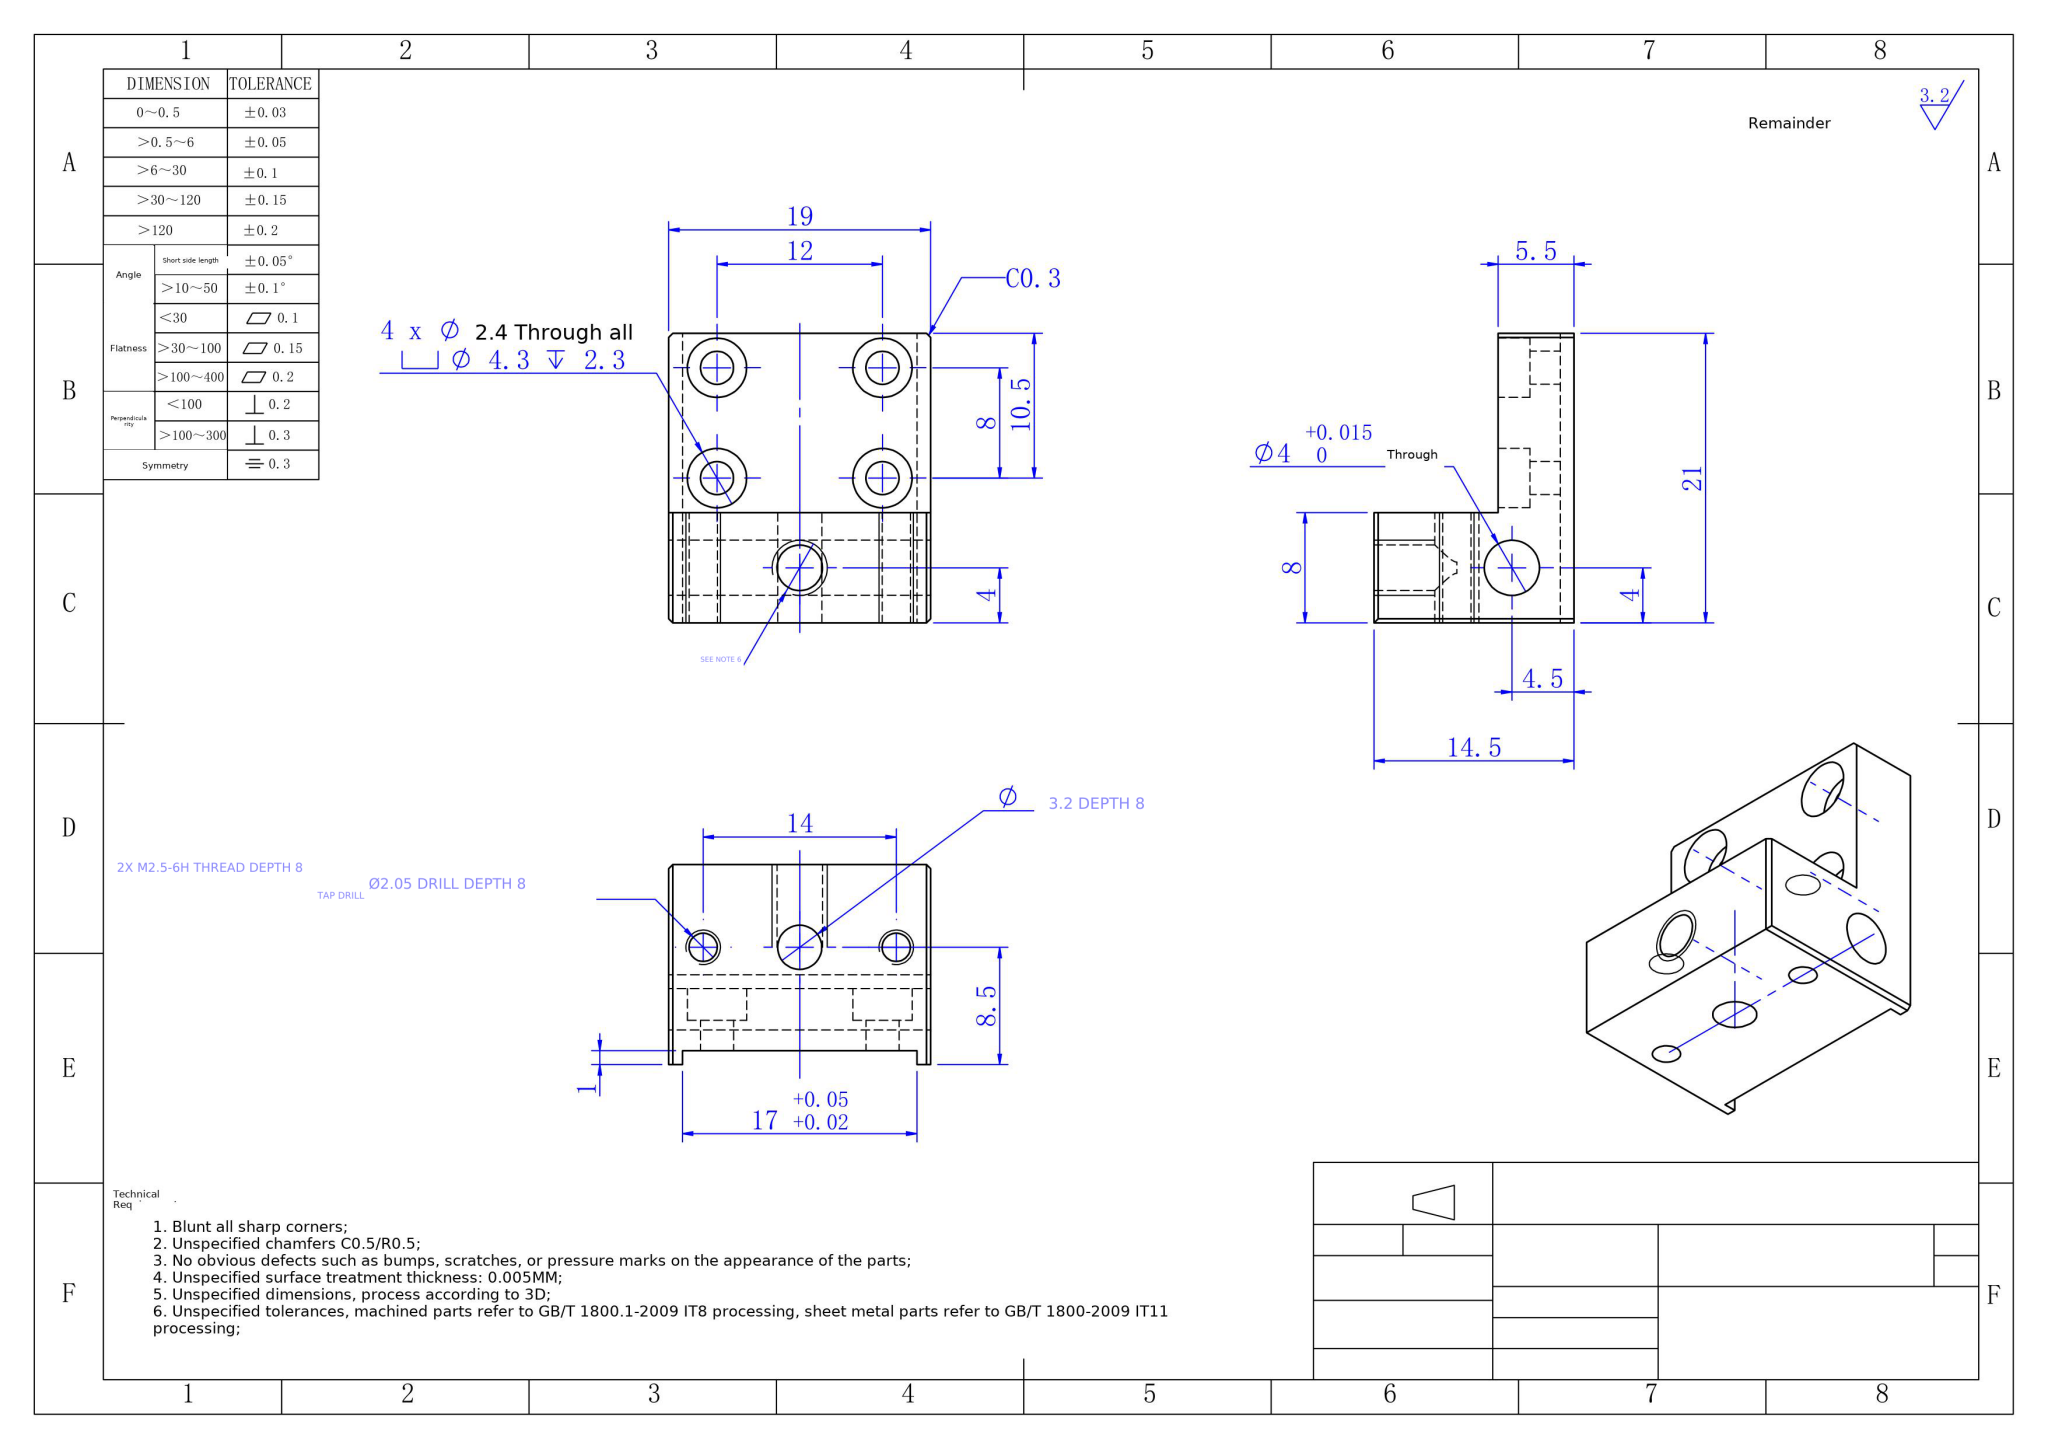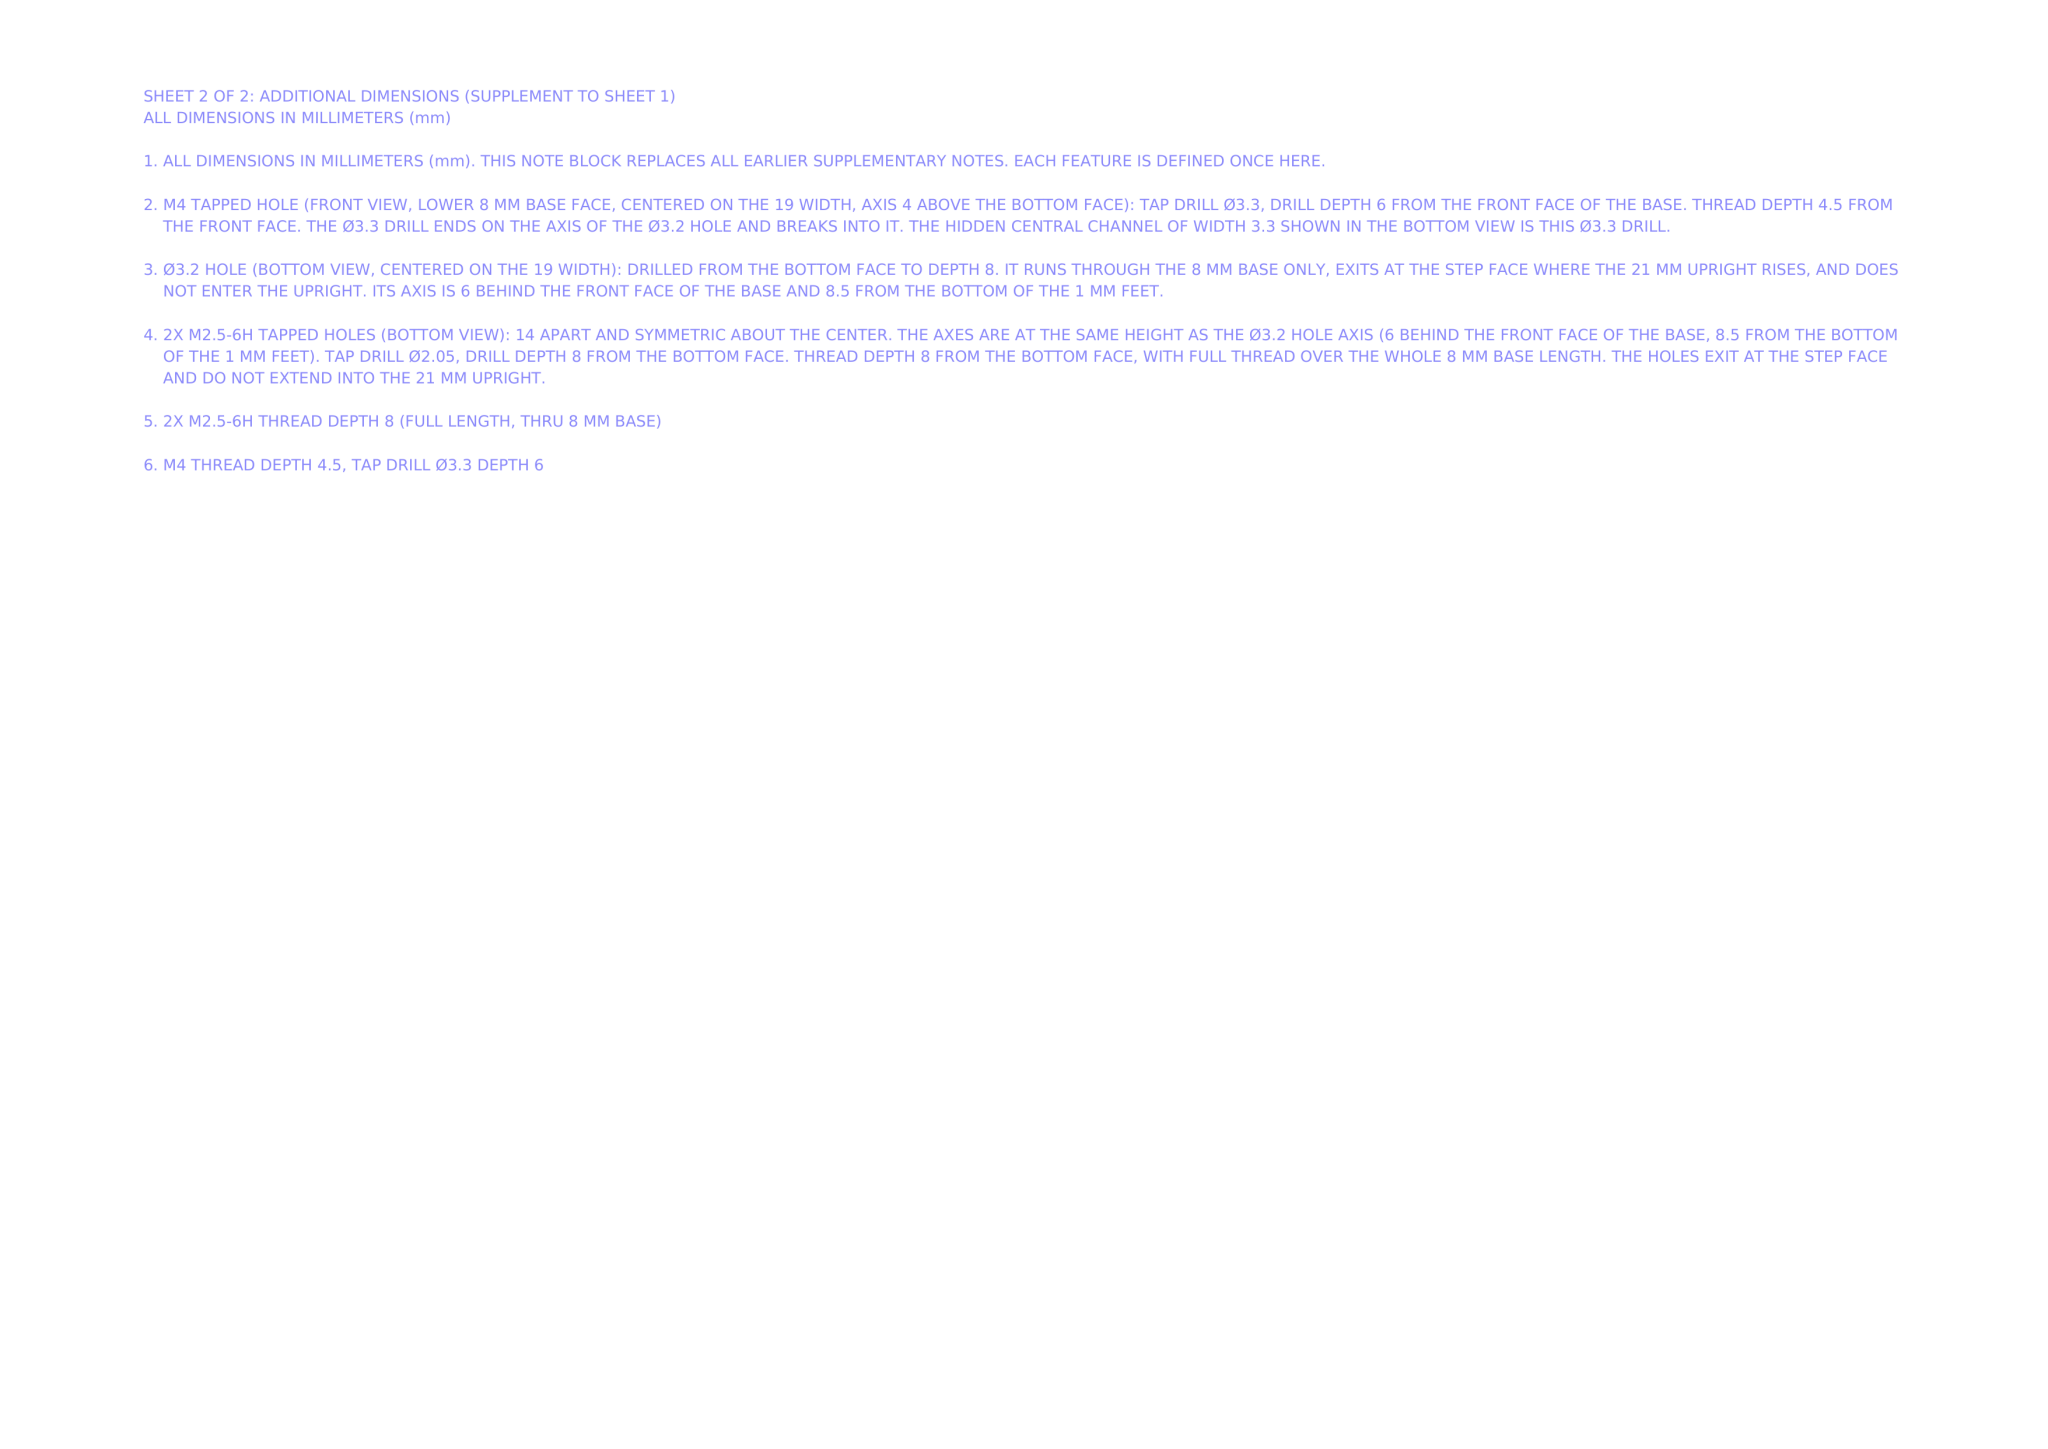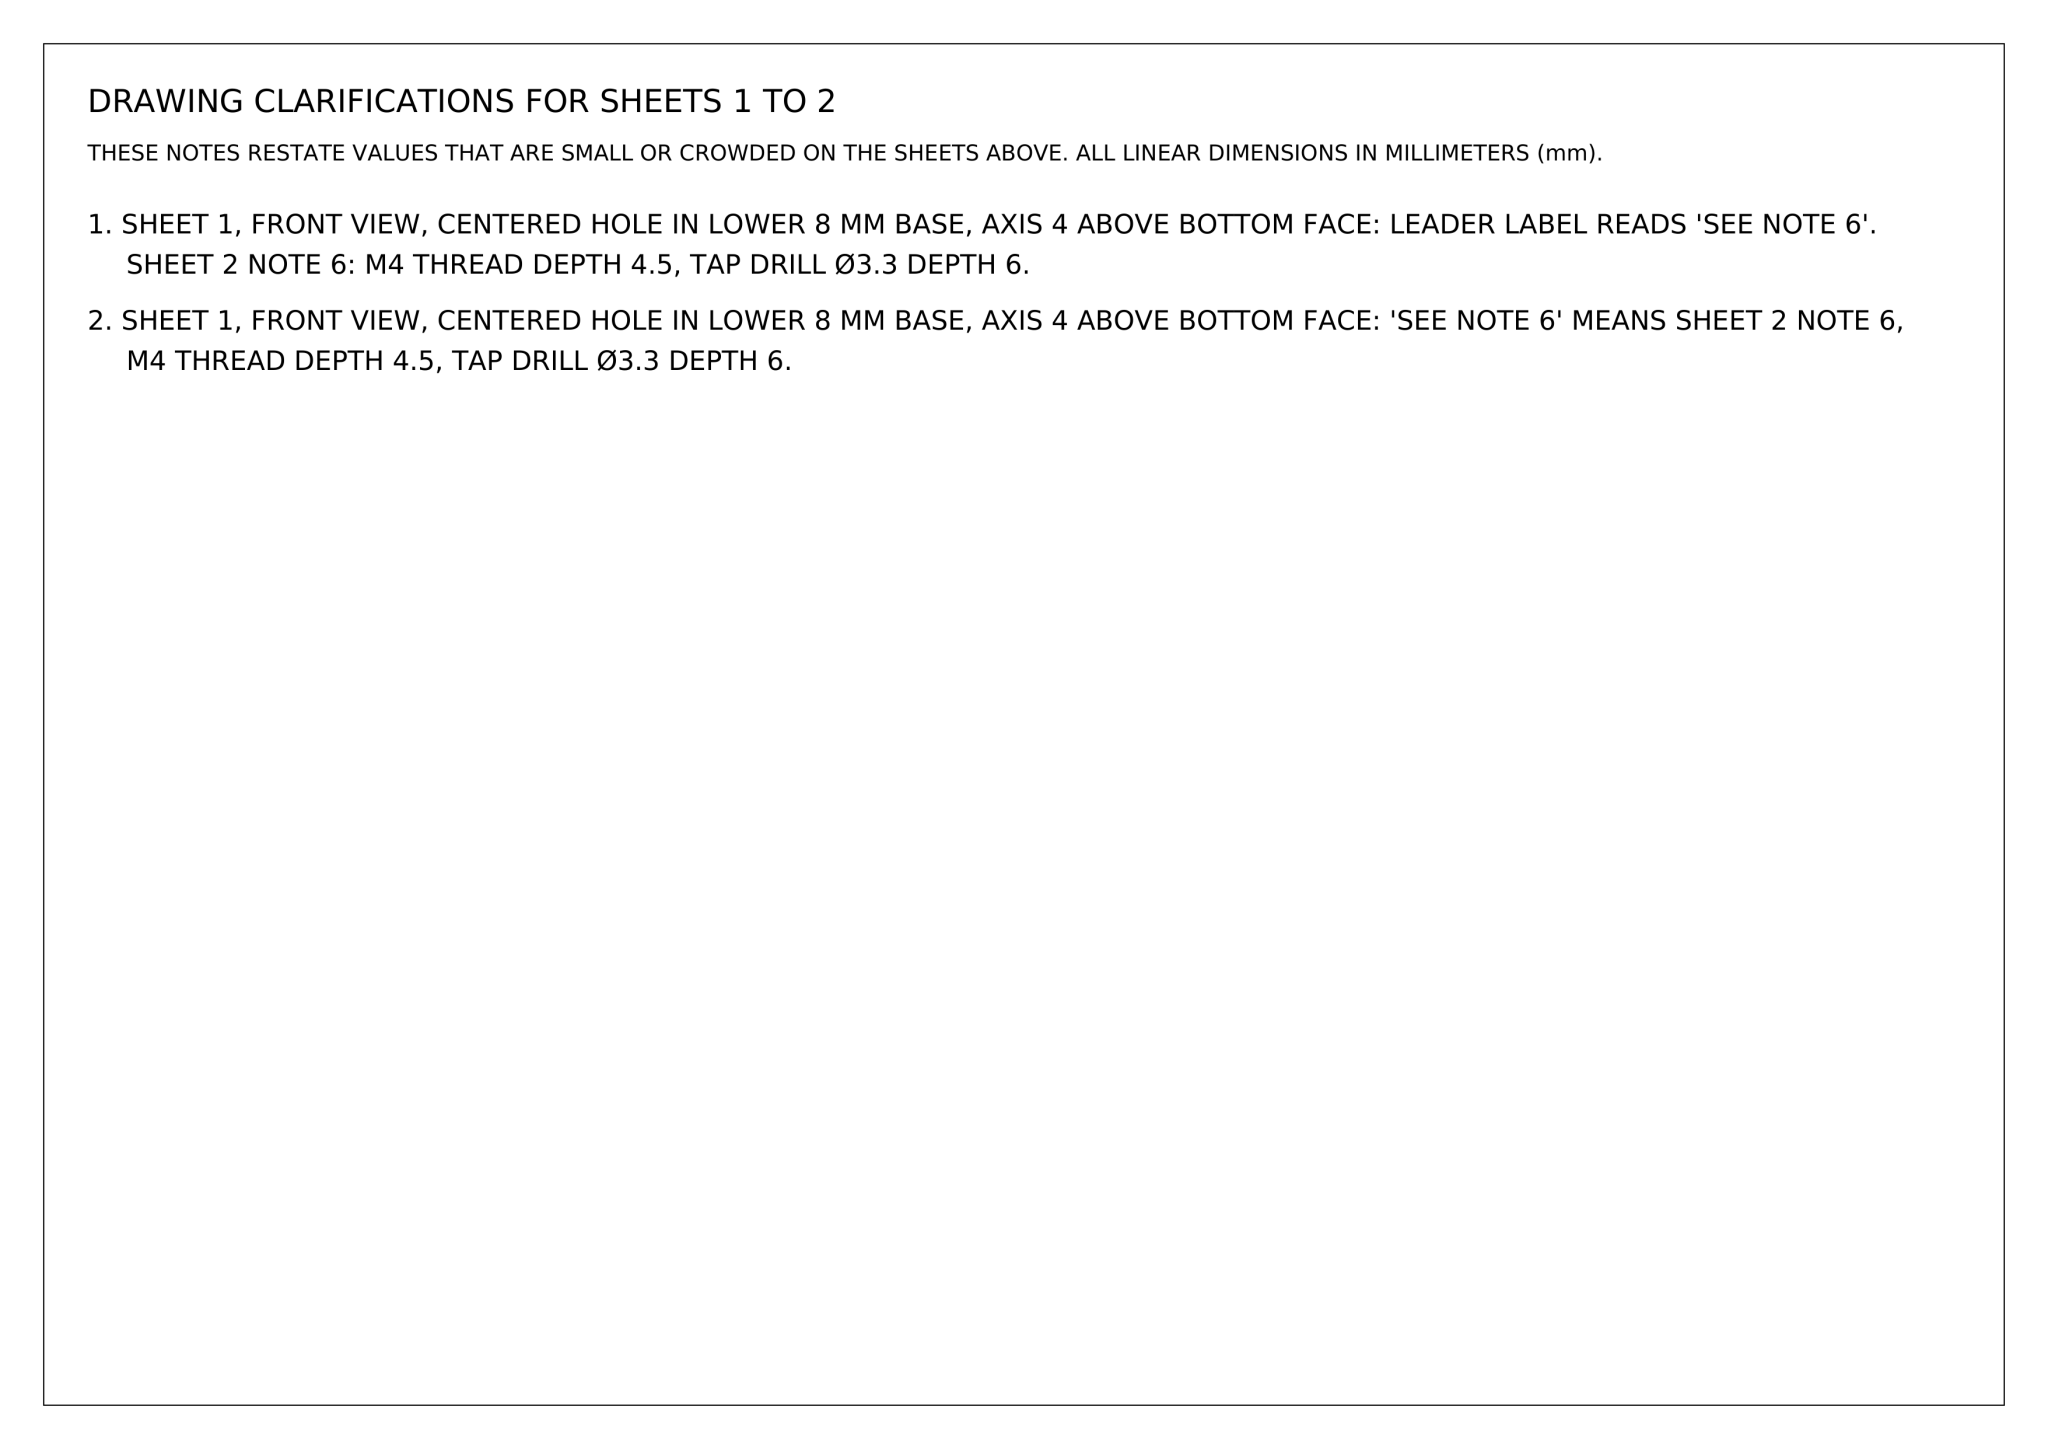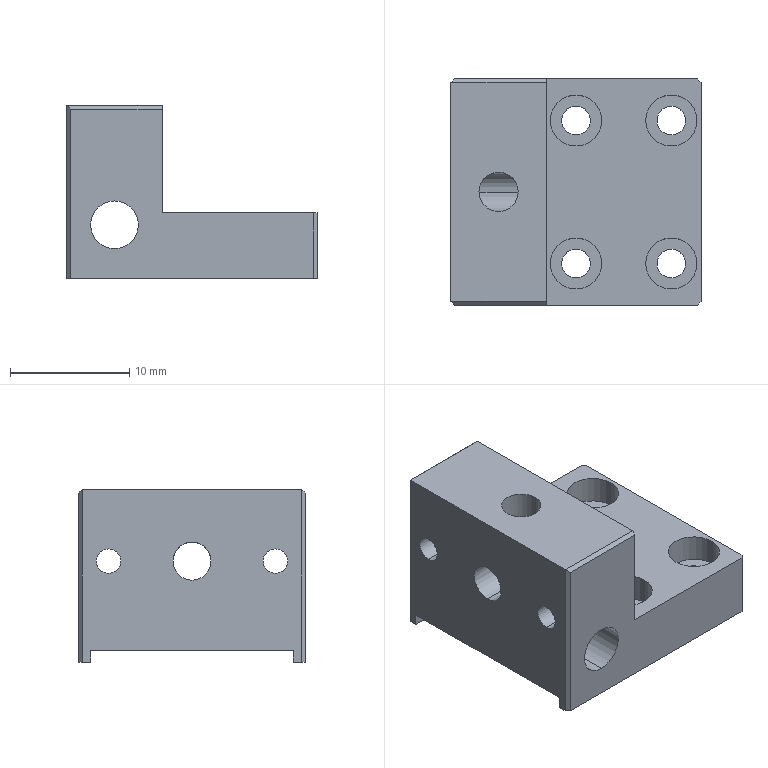Part | NX | mm | 1 solid | 50 faces | box 21 x 19 x 14.5 mm | volume 2634 mm3 | cylinder 26 | plane 24 | commonest cylinder face diameters 4.3 x8 2.4 x8 2.05 x4 3.3 x2 3.2 x2 4 x2